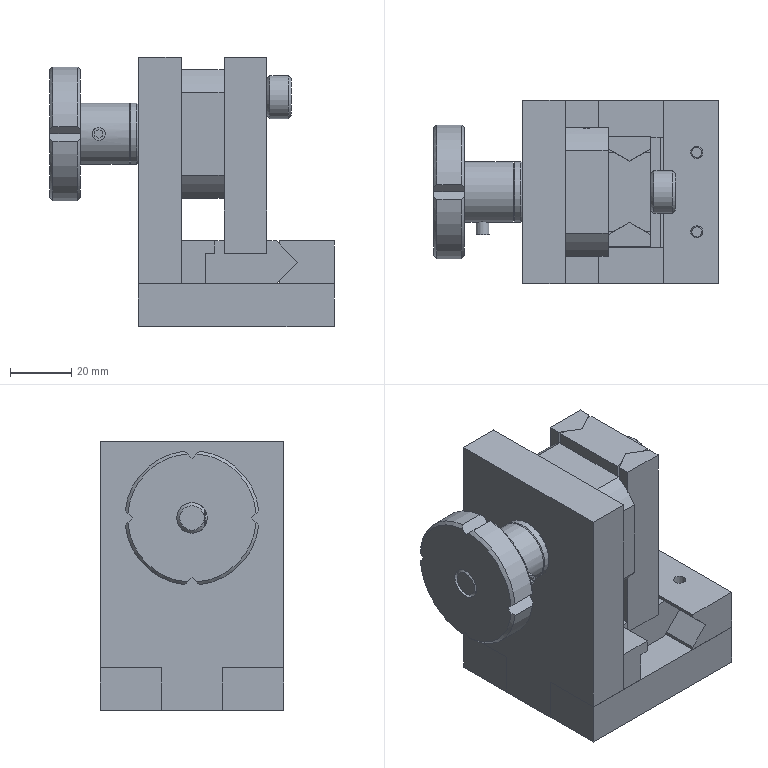Assembly | NX | mm | 26 component files | 26 solids | 438 faces | box 93 x 60 x 88 mm | volume 213179 mm3 | plane 247 | cone 98 | cylinder 86 | torus 7 | commonest cylinder face diameters 4 x18 4.2 x18 8.5 x7 5.5 x7 9.5 x7 1.22 x6 2.3 x6 10 x5
Bill of materials:
unnamed part 1 | 1 |  | Rectangular block with a stepped top. A narrow raised rib runs along one long edge and a wider raised land runs along the other. That opposite side ends in a pointed, V-shaped (male dovetail/prism-like) profile. Three through holes sit in a row between them; the middle hole is larger.
unnamed part 2 | 1 |  | U-shaped prismatic part: two parallel upright arms joined by a solid base, with an open slot between them. Shaded strips on the inner arm faces and the angled arm-end faces suggest a V-shaped groove or chamfered profile running along the inside faces.
unnamed part 3 | 1 |  | Flat annular ring (washer-like disc) with a central circular through hole and small chamfers on the outer edges of both faces.
unnamed part 4 | 1 |  | Rectangular block with a symmetric V-shaped groove cut along each of two opposite faces. A single large circular through hole runs perpendicular to the grooves.
GB-T70.1-2000,M5x16 | 6 |  | Hexagon Socket Head Cap Screw, GB-T 70.1-2000,M5x16
unnamed part 5 | 2 |  | Solid plain cylindrical pin with a chamfered edge at one end; the other end looks square-cut.
unnamed part 6 | 1 |  | Rectangular block with a V-shaped notch (female V) cut into one end face across its full width, and two small circular through holes in the top face.
GB-T120.1-2000,6x24 | 6 |  | Parallel Pin With Internal Thread, GB-T 120.1-2000,6x24
unnamed part 7 | 1 |  | Square plate-like head with chamfered corners, plus a cylindrical shaft sticking out perpendicular from one face. The head has an offset square through opening. The shaft has a chamfered tip and a flat or reduced section along part of its length near the tip.
unnamed part 8 | 1 |  | Flat rectangular plate of uniform thickness with a rectangular notch cut into the middle of one edge. Ten circular through holes are visible: six larger holes near the corners and four smaller holes inboard of them.
unnamed part 9 | 1 |  | Flanged hub: a circular flange with chamfered edges and four small V-shaped notches at 90-degree spacing around its rim, plus a coaxial cylindrical boss. A central through bore runs through both, and a small radial cross hole goes through the boss wall.
GB-T70.1-2000,M5x10 | 1 |  | Hexagon Socket Head Cap Screw, GB-T 70.1-2000,M5x10
unnamed part 10 | 1 |  | Flat rectangular plate with a narrower rectangular tab projecting from the center of one short edge, and one circular through hole near the opposite end.
unnamed part 11 | 1 |  | Long straight bar with an L-shaped (stepped/rabbeted) cross-section along its full length, and two circular through holes in the top face.
unnamed part 12 | 1 |  | Headed cylindrical pin: a straight shaft with a chamfered free end and a larger-diameter cylindrical head with chamfers on both edges. One side view shows a step on the shaft outline, suggesting a flat or reduced section near the free end.
Mates:
1. fix | 1_base_plate 1 component
2. touch align | 2_vertical_plate 1 face | 1_base_plate 1 face
3. touch align | 2_vertical_plate 1 face | 1_base_plate 1 face
4. touch align | 2_vertical_plate 1 face | 1_base_plate 1 face
5. touch align | 2_vertical_plate 1 face | 1_base_plate 1 face
6. touch align | 4_V_guide 1 face | 1_base_plate 1 face
7. touch align | 4_V_guide 1 face | 1_base_plate 1 face
8. touch align | 4_V_guide 1 face | 1_base_plate 1 face
9. touch align | 4_V_guide 1 face | 1_base_plate 1 face
10. touch align | 3_rectangular_guide 1 face | 1_base_plate 1 face
11. touch align | 3_rectangular_guide 1 face | 1_base_plate 1 face
12. touch align | 3_rectangular_guide 1 face | 1_base_plate 1 face
13. touch align | 5_LR_slider 1 face | 3_rectangular_guide 1 face
14. touch align | 6_fork 1 face | 5_LR_slider 1 face
15. touch align | 6_fork 1 face | 5_LR_slider 1 face
16. touch align | 6_fork 1 face | 5_LR_slider 1 face
17. touch align | 14_T70_1_M5x10_cap_screw 1 | 5_LR_slider 1 face
18. touch align | 14_T70_1_M5x10_cap_screw 1 face | 5_LR_slider 1 face
19. touch align | 15_T120_1_M4x24_threaded_dowel_pin 6 face | 5_LR_slider 1 face
20. touch align | 15_T120_1_M4x24_threaded_dowel_pin 5 face | 5_LR_slider 1 face
21. touch align | 15_T120_1_M4x24_threaded_dowel_pin 6 face | 5_LR_slider 1 face
22. touch align | 15_T120_1_M4x24_threaded_dowel_pin 5 face | 5_LR_slider 1 face
23. touch align | 5_LR_slider 1 face | 1_base_plate 1 face
24. touch align | 7_revolving_lift_slider 1 face | 6_fork 1 face
25. parallel | 7_revolving_lift_slider 1 face | 2_vertical_plate 1 face
26. touch align | 8_rotating_shaft 1 face | 2_vertical_plate 1 face
27. touch align | 8_rotating_shaft 1 face | 2_vertical_plate 1 face
28. touch align | 10_handle 1 face | 8_rotating_shaft 1 face
29. touch align | 11_washer 1 face | 8_rotating_shaft 1 face
30. touch align | 11_washer 1 face | 2_vertical_plate 1 face
31. touch align | 10_handle 1 face | 11_washer 1 face
32. touch align | 9_lever 1 face | 7_revolving_lift_slider 1 face
33. touch align | 9_lever 1 face | 7_revolving_lift_slider 1 face
34. touch align | 13_T70_1_M5x14_cap_screw 1 | 1_base_plate 1 face
35. touch align | 13_T70_1_M5x14_cap_screw 2 | 1_base_plate 1 face
36. touch align | 13_T70_1_M5x14_cap_screw 3 | 1_base_plate 1 face
37. touch align | 13_T70_1_M5x14_cap_screw 4 | 1_base_plate 1 face
38. touch align | 13_T70_1_M5x14_cap_screw 6 | 1_base_plate 1 face
39. touch align | 13_T70_1_M5x14_cap_screw 5 | 1_base_plate 1 face
40. touch align | 13_T70_1_M5x14_cap_screw 3 face | 13_T70_1_M5x14_cap_screw 6 face
41. touch align | 13_T70_1_M5x14_cap_screw 5 face | 13_T70_1_M5x14_cap_screw 3 face
42. touch align | 13_T70_1_M5x14_cap_screw 4 face | 13_T70_1_M5x14_cap_screw 3 face
43. touch align | 13_T70_1_M5x14_cap_screw 2 face | 13_T70_1_M5x14_cap_screw 3 face
44. touch align | 13_T70_1_M5x14_cap_screw 1 face | 13_T70_1_M5x14_cap_screw 3 face
45. touch align | 13_T70_1_M5x14_cap_screw 1 face | 1_base_plate 1 face
46. touch align | 15_T120_1_M4x24_threaded_dowel_pin 4 face | 1_base_plate 1 face
47. touch align | 15_T120_1_M4x24_threaded_dowel_pin 1 face | 1_base_plate 1 face
48. touch align | 15_T120_1_M4x24_threaded_dowel_pin 3 face | 1_base_plate 1 face
49. touch align | 15_T120_1_M4x24_threaded_dowel_pin 2 face | 1_base_plate 1 face
50. touch align | 15_T120_1_M4x24_threaded_dowel_pin 1 face | 1_base_plate 1 face
51. touch align | 15_T120_1_M4x24_threaded_dowel_pin 4 face | 1_base_plate 1 face
52. touch align | 15_T120_1_M4x24_threaded_dowel_pin 3 face | 1_base_plate 1 face
53. touch align | 15_T120_1_M4x24_threaded_dowel_pin 2 face | 1_base_plate 1 face
54. touch align | 12_T77_2007_M5x10_flat_set_screw 2 | 10_handle 1 face
55. touch align | 12_T77_2007_M5x10_flat_set_screw 2 face | 8_rotating_shaft 1 face
56. touch align | 12_T77_2007_M5x10_flat_set_screw 1 | 8_rotating_shaft 1 face
57. touch align | 12_T77_2007_M5x10_flat_set_screw 1 face | 9_lever 1 face